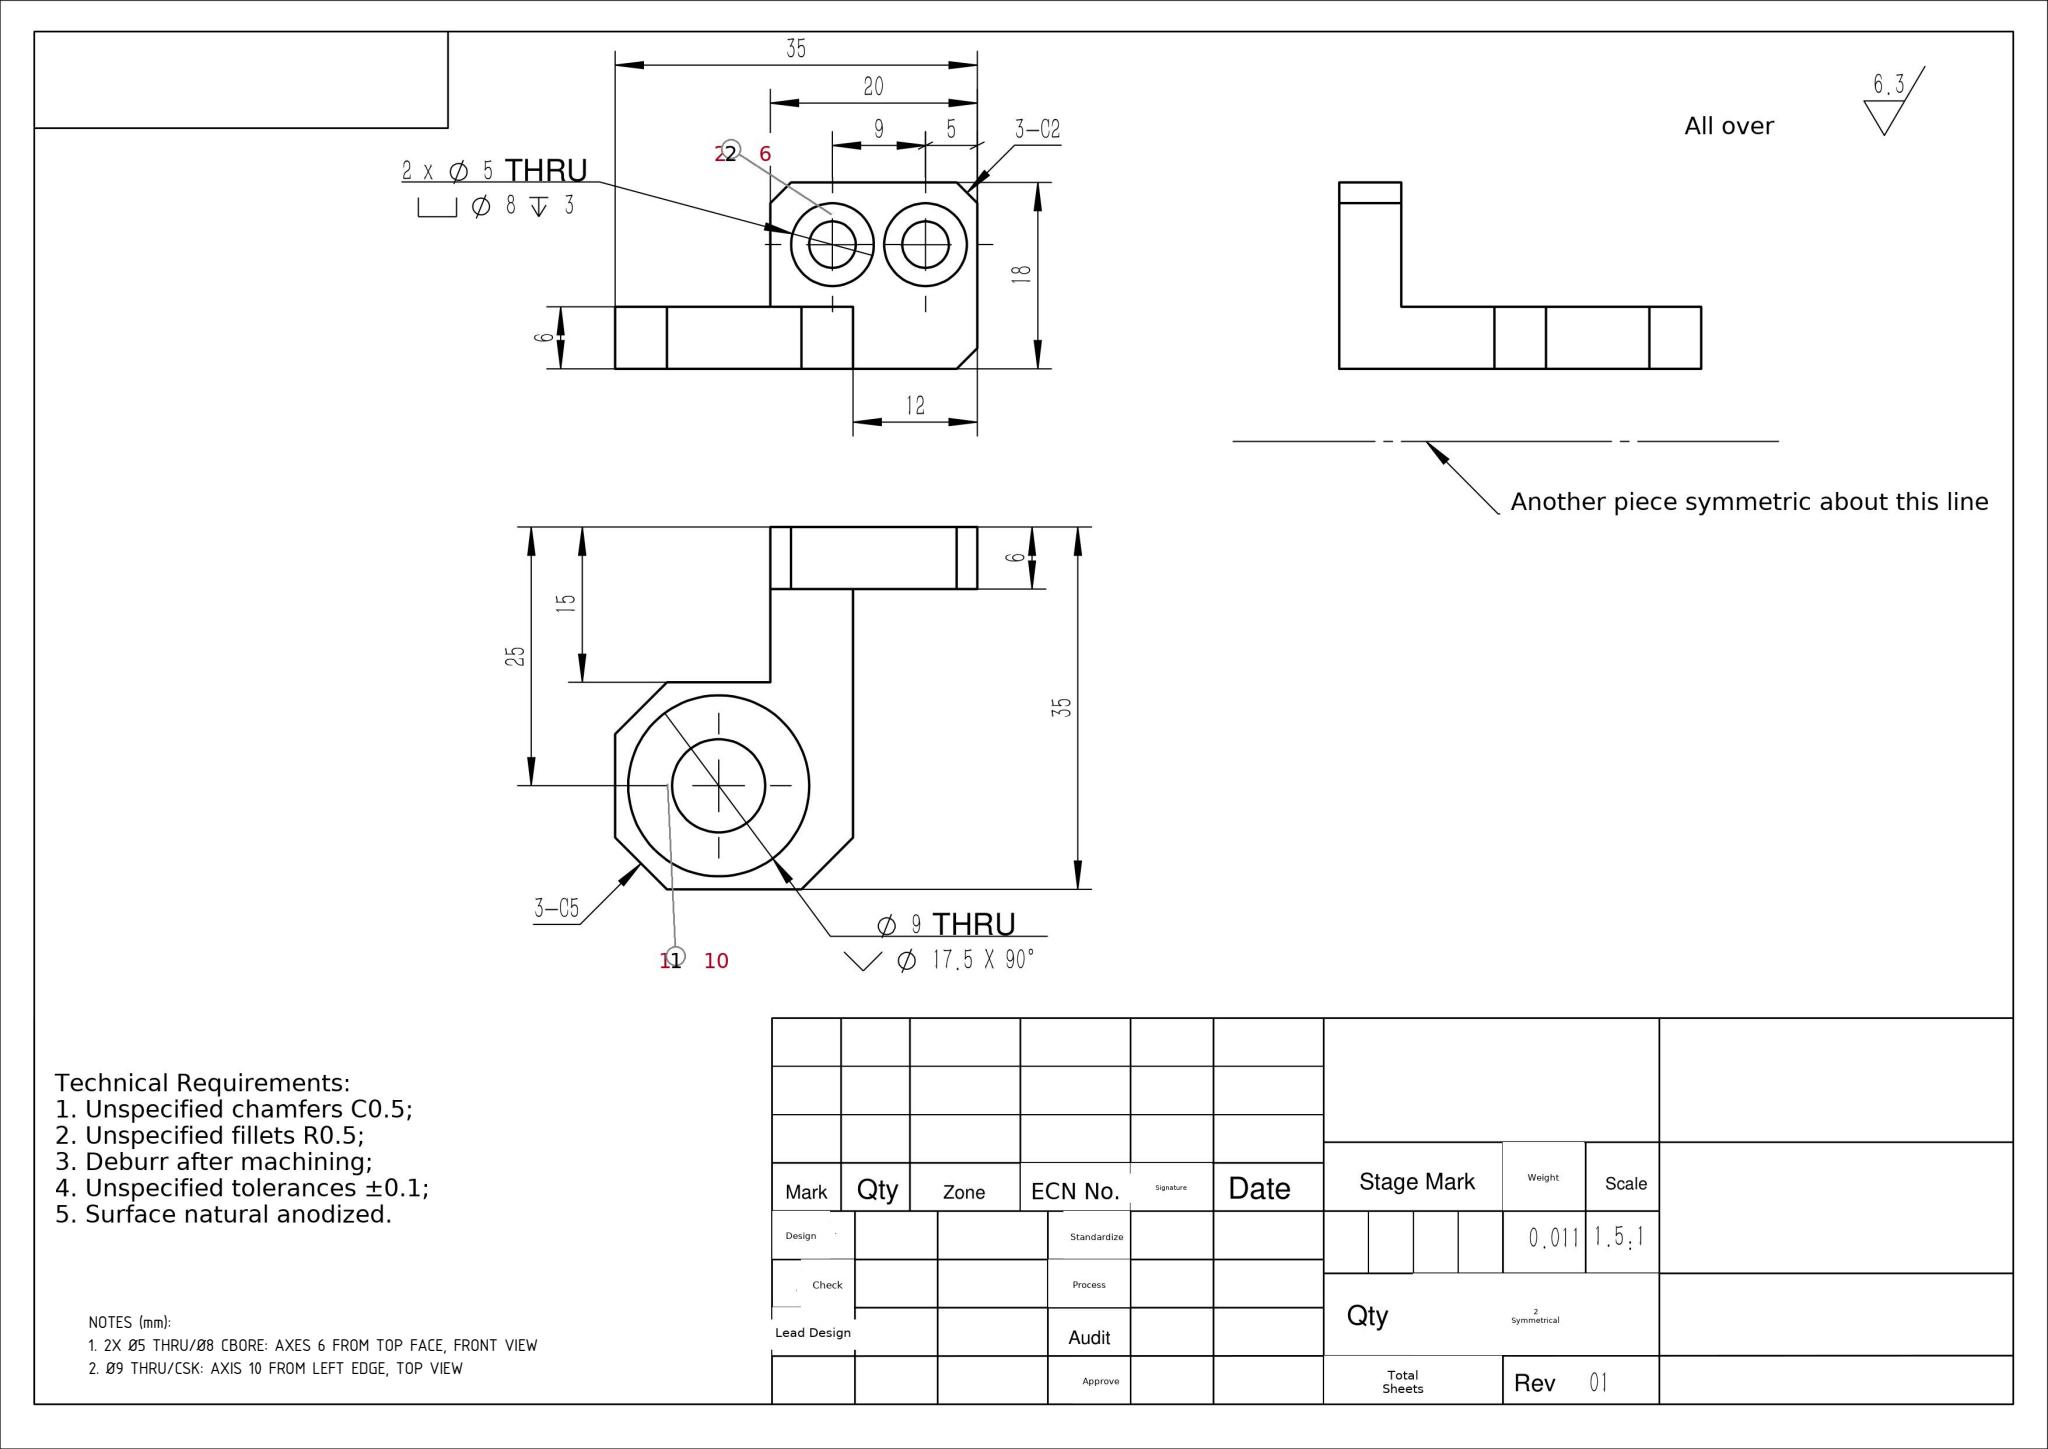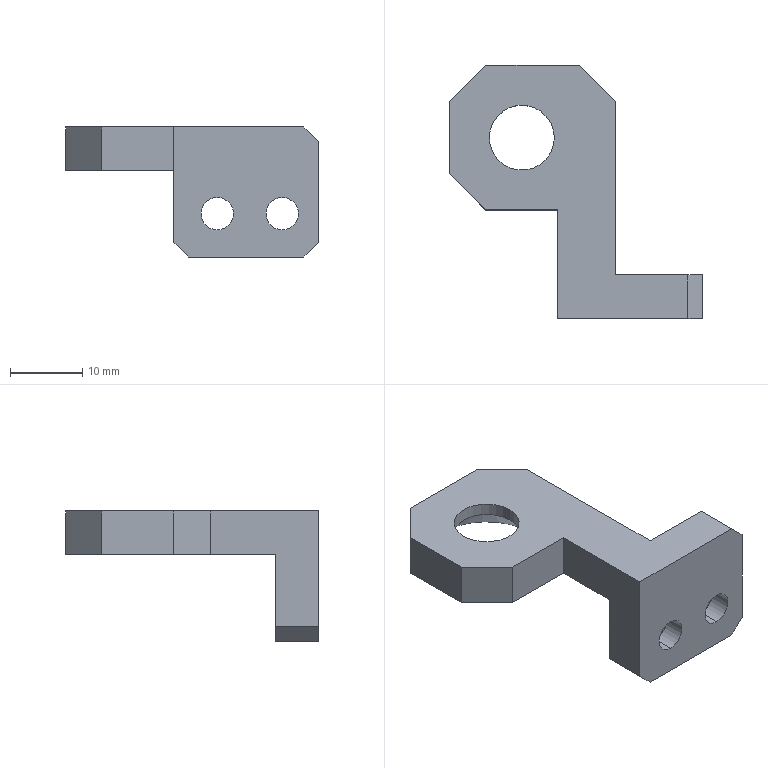Part | SolidWorks | mm | 1 solid | 31 faces | box 35 x 35 x 18 mm | volume 3977 mm3 | plane 19 | cylinder 10 | cone 2 | commonest cylinder face diameters 8 x4 4.5 x4 9 x2
Drawing notes:
2X Ø5 THRU/Ø8 CBORE: AXES 6 FROM TOP FACE, FRONT VIEW | from the solid: Y-axis cyls Ø5/Ø8 at z=6.0 of 18.0 bbox height; top face plane z=0
Ø9 THRU/CSK: AXIS 10 FROM LEFT EDGE, TOP VIEW | from the solid: Z-axis Ø9 cyl at x=10.0 (y=25.0) in 35.0 x 35.0 bbox; left edge plane x=0
build123d program:
from build123d import *

# Parameters (mm, degrees)
SKETCH1_W                                         = 35
SKETCH1_H                                         = 35
BOSS_EXTRUDE1_DEPTH                               = 6
SKETCH2_W                                         = 35
SKETCH2_H                                         = 12
BOSS_EXTRUDE2_DEPTH                               = 6
HOLE_SIZE_ACCORDING_TO_HEXAGON_SOCKET_D           = 4.5
HOLE_SIZE_ACCORDING_TO_HEXAGON_SOCKET_CBORE_D     = 8
HOLE_SIZE_ACCORDING_TO_HEXAGON_SOCKET_CBORE_DEPTH = 3
SKETCH7_W                                         = 15
SKETCH7_H                                         = 15
CUT_EXTRUDE1_DEPTH                                = 31.602
SKETCH8_W                                         = 12
SKETCH8_H                                         = 29
CUT_EXTRUDE2_DEPTH                                = 28.505
CHAMFER1_SIZE                                     = 5
CHAMFER2_SIZE                                     = 2


with BuildPart() as part:
    # Sketch1 → Boss-Extrude1 (new body)
    with BuildSketch(Plane.XY):
        Rectangle(SKETCH1_W, SKETCH1_H)
    extrude(amount=BOSS_EXTRUDE1_DEPTH)

    # Sketch2 → Boss-Extrude2 (add)
    with BuildSketch(Plane.XZ.offset(17.5)):
        with Locations((0, -6)):
            Rectangle(SKETCH2_W, SKETCH2_H)
    extrude(amount=-BOSS_EXTRUDE2_DEPTH)

    # Sketch3 → Hole Size _ according to Phillips_ Raise (revolve, cut)
    with BuildSketch(Plane(origin=(-7.5, 7.5, 0), x_dir=(0, 1, 0), z_dir=(1, 0, 0))):
        Polygon((0, 0), (0, 6), (4.5, 6), (4.5, 4.25), (8.75, 0), align=None)
    revolve(axis=Axis((-7.5, 7.5, -6.35), (0, 0, 1)), mode=Mode.SUBTRACT)

    # Hole Size _ according to_ Hexagon Socket (through all)
    with Locations(Plane(origin=(0, -11.5, 0), x_dir=(1, 0, 0), z_dir=(0, 1, 0))):
        with Locations((3.5, 6), (12.5, 6)):
            CounterBoreHole(HOLE_SIZE_ACCORDING_TO_HEXAGON_SOCKET_D / 2, HOLE_SIZE_ACCORDING_TO_HEXAGON_SOCKET_CBORE_D / 2, HOLE_SIZE_ACCORDING_TO_HEXAGON_SOCKET_CBORE_DEPTH)

    # Sketch7 → Cut-Extrude1 (cut, through all)
    with BuildSketch(Plane(origin=(0, 0, -12), x_dir=(-1, 0, 0), z_dir=(0, 0, -1))):
        with Locations((10, -10)):
            Rectangle(SKETCH7_W, SKETCH7_H)
    extrude(amount=-CUT_EXTRUDE1_DEPTH, mode=Mode.SUBTRACT)

    # Sketch8 → Cut-Extrude2 (cut, through all)
    with BuildSketch(Plane(origin=(0, 0, 0), x_dir=(-1, 0, 0), z_dir=(0, 0, -1))):
        with Locations((-11.5, 3)):
            Rectangle(SKETCH8_W, SKETCH8_H)
    extrude(amount=-CUT_EXTRUDE2_DEPTH, mode=Mode.SUBTRACT)

    # Chamfer1
    chamfer1_edges = [part.edges().sort_by_distance(p)[0] for p in [
        (-17.5, 17.5, 3),
        (-17.5, -2.5, 3),
        (5.5, 17.5, 3),
    ]]
    chamfer(chamfer1_edges, length=CHAMFER1_SIZE)

    # Chamfer2
    chamfer2_edges = [part.edges().sort_by_distance(p)[0] for p in [
        (17.5, -14.5, -12),
        (-2.5, -14.5, -12),
        (17.5, -14.5, 6),
    ]]
    chamfer(chamfer2_edges, length=CHAMFER2_SIZE)


solid = part.part
STEP:
#1=CARTESIAN_POINT('',(3.5,-14.5,-10.));
#2=VERTEX_POINT('',#1);
#3=CARTESIAN_POINT('',(3.5,-14.5,-2.));
#4=VERTEX_POINT('',#3);
#5=CARTESIAN_POINT('',(3.5,-14.5,-6.));
#6=DIRECTION('',(0.,1.,0.));
#7=DIRECTION('',(0.,0.,1.));
#8=AXIS2_PLACEMENT_3D('',#5,#6,#7);
#9=CIRCLE('',#8,4.);
#10=EDGE_CURVE('',#2,#4,#9,.T.);
#11=ORIENTED_EDGE('',*,*,#10,.F.);
#12=CARTESIAN_POINT('',(3.5,-11.5,-10.));
#13=VERTEX_POINT('',#12);
#14=CARTESIAN_POINT('',(3.5,-11.5,-10.));
#15=DIRECTION('',(0.,1.,0.));
#16=VECTOR('',#15,1000.);
#17=LINE('',#14,#16);
#18=EDGE_CURVE('',#2,#13,#17,.T.);
#19=ORIENTED_EDGE('',*,*,#18,.T.);
#20=CARTESIAN_POINT('',(3.5,-11.5,-2.));
#21=VERTEX_POINT('',#20);
#22=CARTESIAN_POINT('',(3.5,-11.5,-6.));
#23=DIRECTION('',(0.,1.,0.));
#24=DIRECTION('',(0.,0.,1.));
#25=AXIS2_PLACEMENT_3D('',#22,#23,#24);
#26=CIRCLE('',#25,4.);
#27=EDGE_CURVE('',#13,#21,#26,.T.);
#28=ORIENTED_EDGE('',*,*,#27,.T.);
#29=CARTESIAN_POINT('',(3.5,-11.5,-2.));
#30=DIRECTION('',(0.,1.,0.));
#31=VECTOR('',#30,1000.);
#32=LINE('',#29,#31);
#33=EDGE_CURVE('',#4,#21,#32,.T.);
#34=ORIENTED_EDGE('',*,*,#33,.F.);
#35=EDGE_LOOP('',(#11,#19,#28,#34));
#36=FACE_OUTER_BOUND('',#35,.T.);
#37=CARTESIAN_POINT('',(3.5,-11.5,-6.));
#38=DIRECTION('',(0.,1.,0.));
#39=DIRECTION('',(0.,0.,1.));
#40=AXIS2_PLACEMENT_3D('',#37,#38,#39);
#41=CYLINDRICAL_SURFACE('',#40,4.);
#42=ADVANCED_FACE('',(#36),#41,.F.);
#43=CARTESIAN_POINT('',(3.5,-17.5,-8.25));
#44=VERTEX_POINT('',#43);
#45=CARTESIAN_POINT('',(3.5,-17.5,-3.75));
#46=VERTEX_POINT('',#45);
#47=CARTESIAN_POINT('',(3.5,-17.5,-6.));
#48=DIRECTION('',(0.,1.,0.));
#49=DIRECTION('',(0.,0.,1.));
#50=AXIS2_PLACEMENT_3D('',#47,#48,#49);
#51=CIRCLE('',#50,2.25);
#52=EDGE_CURVE('',#44,#46,#51,.T.);
#53=ORIENTED_EDGE('',*,*,#52,.F.);
#54=CARTESIAN_POINT('',(3.5,-14.5,-8.25));
#55=VERTEX_POINT('',#54);
#56=CARTESIAN_POINT('',(3.5,-11.5,-8.25));
#57=DIRECTION('',(0.,1.,0.));
#58=VECTOR('',#57,1000.);
#59=LINE('',#56,#58);
#60=EDGE_CURVE('',#44,#55,#59,.T.);
#61=ORIENTED_EDGE('',*,*,#60,.T.);
#62=CARTESIAN_POINT('',(3.5,-14.5,-3.75));
#63=VERTEX_POINT('',#62);
#64=CARTESIAN_POINT('',(3.5,-14.5,-6.));
#65=DIRECTION('',(0.,1.,0.));
#66=DIRECTION('',(0.,0.,1.));
#67=AXIS2_PLACEMENT_3D('',#64,#65,#66);
#68=CIRCLE('',#67,2.25);
#69=EDGE_CURVE('',#55,#63,#68,.T.);
#70=ORIENTED_EDGE('',*,*,#69,.T.);
#71=CARTESIAN_POINT('',(3.5,-11.5,-3.75));
#72=DIRECTION('',(0.,1.,0.));
#73=VECTOR('',#72,1000.);
#74=LINE('',#71,#73);
#75=EDGE_CURVE('',#46,#63,#74,.T.);
#76=ORIENTED_EDGE('',*,*,#75,.F.);
#77=EDGE_LOOP('',(#53,#61,#70,#76));
#78=FACE_OUTER_BOUND('',#77,.T.);
#79=CARTESIAN_POINT('',(3.5,-11.5,-6.));
#80=DIRECTION('',(0.,1.,0.));
#81=DIRECTION('',(0.,0.,1.));
#82=AXIS2_PLACEMENT_3D('',#79,#80,#81);
#83=CYLINDRICAL_SURFACE('',#82,2.25);
#84=ADVANCED_FACE('',(#78),#83,.F.);
#85=CARTESIAN_POINT('',(12.5,-14.5,-10.));
#86=VERTEX_POINT('',#85);
#87=CARTESIAN_POINT('',(12.5,-14.5,-2.));
#88=VERTEX_POINT('',#87);
#89=CARTESIAN_POINT('',(12.5,-14.5,-6.));
#90=DIRECTION('',(0.,1.,0.));
#91=DIRECTION('',(0.,0.,1.));
#92=AXIS2_PLACEMENT_3D('',#89,#90,#91);
#93=CIRCLE('',#92,4.);
#94=EDGE_CURVE('',#86,#88,#93,.T.);
#95=ORIENTED_EDGE('',*,*,#94,.F.);
#96=CARTESIAN_POINT('',(12.5,-11.5,-10.));
#97=VERTEX_POINT('',#96);
#98=CARTESIAN_POINT('',(12.5,-11.5,-10.));
#99=DIRECTION('',(0.,1.,0.));
#100=VECTOR('',#99,1000.);
#101=LINE('',#98,#100);
#102=EDGE_CURVE('',#86,#97,#101,.T.);
#103=ORIENTED_EDGE('',*,*,#102,.T.);
#104=CARTESIAN_POINT('',(12.5,-11.5,-2.));
#105=VERTEX_POINT('',#104);
#106=CARTESIAN_POINT('',(12.5,-11.5,-6.));
#107=DIRECTION('',(0.,1.,0.));
#108=DIRECTION('',(0.,0.,1.));
#109=AXIS2_PLACEMENT_3D('',#106,#107,#108);
#110=CIRCLE('',#109,4.);
#111=EDGE_CURVE('',#97,#105,#110,.T.);
#112=ORIENTED_EDGE('',*,*,#111,.T.);
#113=CARTESIAN_POINT('',(12.5,-11.5,-2.));
#114=DIRECTION('',(0.,1.,0.));
#115=VECTOR('',#114,1000.);
#116=LINE('',#113,#115);
#117=EDGE_CURVE('',#88,#105,#116,.T.);
#118=ORIENTED_EDGE('',*,*,#117,.F.);
#119=EDGE_LOOP('',(#95,#103,#112,#118));
#120=FACE_OUTER_BOUND('',#119,.T.);
#121=CARTESIAN_POINT('',(12.5,-11.5,-6.));
#122=DIRECTION('',(0.,1.,0.));
#123=DIRECTION('',(0.,0.,1.));
#124=AXIS2_PLACEMENT_3D('',#121,#122,#123);
#125=CYLINDRICAL_SURFACE('',#124,4.);
#126=ADVANCED_FACE('',(#120),#125,.F.);
#127=CARTESIAN_POINT('',(12.5,-17.5,-8.25));
#128=VERTEX_POINT('',#127);
#129=CARTESIAN_POINT('',(12.5,-17.5,-3.75));
#130=VERTEX_POINT('',#129);
#131=CARTESIAN_POINT('',(12.5,-17.5,-6.));
#132=DIRECTION('',(0.,1.,0.));
#133=DIRECTION('',(0.,0.,1.));
#134=AXIS2_PLACEMENT_3D('',#131,#132,#133);
#135=CIRCLE('',#134,2.25);
#136=EDGE_CURVE('',#128,#130,#135,.T.);
#137=ORIENTED_EDGE('',*,*,#136,.F.);
#138=CARTESIAN_POINT('',(12.5,-14.5,-8.25));
#139=VERTEX_POINT('',#138);
#140=CARTESIAN_POINT('',(12.5,-11.5,-8.25));
#141=DIRECTION('',(0.,1.,0.));
#142=VECTOR('',#141,1000.);
#143=LINE('',#140,#142);
#144=EDGE_CURVE('',#128,#139,#143,.T.);
#145=ORIENTED_EDGE('',*,*,#144,.T.);
#146=CARTESIAN_POINT('',(12.5,-14.5,-3.75));
#147=VERTEX_POINT('',#146);
#148=CARTESIAN_POINT('',(12.5,-14.5,-6.));
#149=DIRECTION('',(0.,1.,0.));
#150=DIRECTION('',(0.,0.,1.));
#151=AXIS2_PLACEMENT_3D('',#148,#149,#150);
#152=CIRCLE('',#151,2.25);
#153=EDGE_CURVE('',#139,#147,#152,.T.);
#154=ORIENTED_EDGE('',*,*,#153,.T.);
#155=CARTESIAN_POINT('',(12.5,-11.5,-3.75));
#156=DIRECTION('',(0.,1.,0.));
#157=VECTOR('',#156,1000.);
#158=LINE('',#155,#157);
#159=EDGE_CURVE('',#130,#147,#158,.T.);
#160=ORIENTED_EDGE('',*,*,#159,.F.);
#161=EDGE_LOOP('',(#137,#145,#154,#160));
#162=FACE_OUTER_BOUND('',#161,.T.);
#163=CARTESIAN_POINT('',(12.5,-11.5,-6.));
#164=DIRECTION('',(0.,1.,0.));
#165=DIRECTION('',(0.,0.,1.));
#166=AXIS2_PLACEMENT_3D('',#163,#164,#165);
#167=CYLINDRICAL_SURFACE('',#166,2.25);
#168=ADVANCED_FACE('',(#162),#167,.F.);
#169=CARTESIAN_POINT('',(-3.,7.5,4.25));
#170=VERTEX_POINT('',#169);
#171=CARTESIAN_POINT('',(-12.,7.5,4.25));
#172=VERTEX_POINT('',#171);
#173=CARTESIAN_POINT('',(-7.5,7.5,4.25));
#174=DIRECTION('',(0.,0.,-1.));
#175=DIRECTION('',(-1.,0.,0.));
#176=AXIS2_PLACEMENT_3D('',#173,#174,#175);
#177=CIRCLE('',#176,4.5);
#178=EDGE_CURVE('',#170,#172,#177,.T.);
#179=ORIENTED_EDGE('',*,*,#178,.F.);
#180=CARTESIAN_POINT('',(1.25,7.5,-0.));
#181=VERTEX_POINT('',#180);
#182=CARTESIAN_POINT('',(1.25,7.5,-0.));
#183=DIRECTION('',(0.7071,0.,-0.7071));
#184=VECTOR('',#183,1000.);
#185=LINE('',#182,#184);
#186=EDGE_CURVE('',#170,#181,#185,.T.);
#187=ORIENTED_EDGE('',*,*,#186,.T.);
#188=CARTESIAN_POINT('',(-16.25,7.5,-0.));
#189=VERTEX_POINT('',#188);
#190=CARTESIAN_POINT('',(-7.5,7.5,-0.));
#191=DIRECTION('',(0.,0.,-1.));
#192=DIRECTION('',(-1.,0.,0.));
#193=AXIS2_PLACEMENT_3D('',#190,#191,#192);
#194=CIRCLE('',#193,8.75);
#195=EDGE_CURVE('',#181,#189,#194,.T.);
#196=ORIENTED_EDGE('',*,*,#195,.T.);
#197=CARTESIAN_POINT('',(-16.25,7.5,-0.));
#198=DIRECTION('',(-0.7071,0.,-0.7071));
#199=VECTOR('',#198,1000.);
#200=LINE('',#197,#199);
#201=EDGE_CURVE('',#172,#189,#200,.T.);
#202=ORIENTED_EDGE('',*,*,#201,.F.);
#203=EDGE_LOOP('',(#179,#187,#196,#202));
#204=FACE_OUTER_BOUND('',#203,.T.);
#205=CARTESIAN_POINT('',(-7.5,7.5,-0.));
#206=DIRECTION('',(0.,0.,-1.));
#207=DIRECTION('',(-1.,0.,0.));
#208=AXIS2_PLACEMENT_3D('',#205,#206,#207);
#209=CONICAL_SURFACE('',#208,8.75,0.7854);
#210=ADVANCED_FACE('',(#204),#209,.F.);
#211=CARTESIAN_POINT('',(-3.,7.5,6.));
#212=VERTEX_POINT('',#211);
#213=CARTESIAN_POINT('',(-12.,7.5,6.));
#214=VERTEX_POINT('',#213);
#215=CARTESIAN_POINT('',(-7.5,7.5,6.));
#216=DIRECTION('',(0.,0.,-1.));
#217=DIRECTION('',(-1.,0.,0.));
#218=AXIS2_PLACEMENT_3D('',#215,#216,#217);
#219=CIRCLE('',#218,4.5);
#220=EDGE_CURVE('',#212,#214,#219,.T.);
#221=ORIENTED_EDGE('',*,*,#220,.F.);
#222=CARTESIAN_POINT('',(-3.,7.5,0.));
#223=DIRECTION('',(0.,0.,-1.));
#224=VECTOR('',#223,1000.);
#225=LINE('',#222,#224);
#226=EDGE_CURVE('',#212,#170,#225,.T.);
#227=ORIENTED_EDGE('',*,*,#226,.T.);
#228=ORIENTED_EDGE('',*,*,#178,.T.);
#229=CARTESIAN_POINT('',(-12.,7.5,0.));
#230=DIRECTION('',(0.,0.,-1.));
#231=VECTOR('',#230,1000.);
#232=LINE('',#229,#231);
#233=EDGE_CURVE('',#214,#172,#232,.T.);
#234=ORIENTED_EDGE('',*,*,#233,.F.);
#235=EDGE_LOOP('',(#221,#227,#228,#234));
#236=FACE_OUTER_BOUND('',#235,.T.);
#237=CARTESIAN_POINT('',(-7.5,7.5,0.));
#238=DIRECTION('',(0.,0.,-1.));
#239=DIRECTION('',(-1.,0.,0.));
#240=AXIS2_PLACEMENT_3D('',#237,#238,#239);
#241=CYLINDRICAL_SURFACE('',#240,4.5);
#242=ADVANCED_FACE('',(#236),#241,.F.);
#243=CARTESIAN_POINT('',(-17.5,12.5,0.));
#244=VERTEX_POINT('',#243);
#245=CARTESIAN_POINT('',(-17.5,2.5,0.));
#246=VERTEX_POINT('',#245);
#247=CARTESIAN_POINT('',(-17.5,-17.5,0.));
#248=DIRECTION('',(0.,-1.,0.));
#249=VECTOR('',#248,1000.);
#250=LINE('',#247,#249);
#251=EDGE_CURVE('',#244,#246,#250,.T.);
#252=ORIENTED_EDGE('',*,*,#251,.T.);
#253=CARTESIAN_POINT('',(-17.5,2.5,6.));
#254=VERTEX_POINT('',#253);
#255=CARTESIAN_POINT('',(-17.5,2.5,6.));
#256=DIRECTION('',(0.,0.,1.));
#257=VECTOR('',#256,1000.);
#258=LINE('',#255,#257);
#259=EDGE_CURVE('',#246,#254,#258,.T.);
#260=ORIENTED_EDGE('',*,*,#259,.T.);
#261=CARTESIAN_POINT('',(-17.5,12.5,6.));
#262=VERTEX_POINT('',#261);
#263=CARTESIAN_POINT('',(-17.5,-17.5,6.));
#264=DIRECTION('',(0.,-1.,0.));
#265=VECTOR('',#264,1000.);
#266=LINE('',#263,#265);
#267=EDGE_CURVE('',#262,#254,#266,.T.);
#268=ORIENTED_EDGE('',*,*,#267,.F.);
#269=CARTESIAN_POINT('',(-17.5,12.5,6.));
#270=DIRECTION('',(0.,0.,-1.));
#271=VECTOR('',#270,1000.);
#272=LINE('',#269,#271);
#273=EDGE_CURVE('',#262,#244,#272,.T.);
#274=ORIENTED_EDGE('',*,*,#273,.T.);
#275=EDGE_LOOP('',(#252,#260,#268,#274));
#276=FACE_OUTER_BOUND('',#275,.T.);
#277=CARTESIAN_POINT('',(-17.5,-17.5,6.));
#278=DIRECTION('',(1.,0.,0.));
#279=DIRECTION('',(0.,0.,-1.));
#280=AXIS2_PLACEMENT_3D('',#277,#278,#279);
#281=PLANE('',#280);
#282=ADVANCED_FACE('',(#276),#281,.F.);
#283=CARTESIAN_POINT('',(3.5,-17.5,-6.));
#284=DIRECTION('',(0.,1.,0.));
#285=DIRECTION('',(0.,0.,1.));
#286=AXIS2_PLACEMENT_3D('',#283,#284,#285);
#287=CIRCLE('',#286,2.25);
#288=EDGE_CURVE('',#46,#44,#287,.T.);
#289=ORIENTED_EDGE('',*,*,#288,.T.);
#290=ORIENTED_EDGE('',*,*,#52,.T.);
#291=EDGE_LOOP('',(#289,#290));
#292=FACE_BOUND('',#291,.T.);
#293=CARTESIAN_POINT('',(12.5,-17.5,-6.));
#294=DIRECTION('',(0.,1.,0.));
#295=DIRECTION('',(0.,0.,1.));
#296=AXIS2_PLACEMENT_3D('',#293,#294,#295);
#297=CIRCLE('',#296,2.25);
#298=EDGE_CURVE('',#130,#128,#297,.T.);
#299=ORIENTED_EDGE('',*,*,#298,.T.);
#300=ORIENTED_EDGE('',*,*,#136,.T.);
#301=EDGE_LOOP('',(#299,#300));
#302=FACE_BOUND('',#301,.T.);
#303=CARTESIAN_POINT('',(17.5,-17.5,4.));
#304=VERTEX_POINT('',#303);
#305=CARTESIAN_POINT('',(17.5,-17.5,-10.));
#306=VERTEX_POINT('',#305);
#307=CARTESIAN_POINT('',(17.5,-17.5,6.));
#308=DIRECTION('',(0.,0.,-1.));
#309=VECTOR('',#308,1000.);
#310=LINE('',#307,#309);
#311=EDGE_CURVE('',#304,#306,#310,.T.);
#312=ORIENTED_EDGE('',*,*,#311,.F.);
#313=CARTESIAN_POINT('',(15.5,-17.5,6.));
#314=VERTEX_POINT('',#313);
#315=CARTESIAN_POINT('',(15.5,-17.5,6.));
#316=DIRECTION('',(-0.7071,0.,0.7071));
#317=VECTOR('',#316,1000.);
#318=LINE('',#315,#317);
#319=EDGE_CURVE('',#304,#314,#318,.T.);
#320=ORIENTED_EDGE('',*,*,#319,.T.);
#321=CARTESIAN_POINT('',(-2.5,-17.5,6.));
#322=VERTEX_POINT('',#321);
#323=CARTESIAN_POINT('',(17.5,-17.5,6.));
#324=DIRECTION('',(1.,0.,0.));
#325=VECTOR('',#324,1000.);
#326=LINE('',#323,#325);
#327=EDGE_CURVE('',#322,#314,#326,.T.);
#328=ORIENTED_EDGE('',*,*,#327,.F.);
#329=CARTESIAN_POINT('',(-2.5,-17.5,-10.));
#330=VERTEX_POINT('',#329);
#331=CARTESIAN_POINT('',(-2.5,-17.5,6.));
#332=DIRECTION('',(0.,0.,-1.));
#333=VECTOR('',#332,1000.);
#334=LINE('',#331,#333);
#335=EDGE_CURVE('',#322,#330,#334,.T.);
#336=ORIENTED_EDGE('',*,*,#335,.T.);
#337=CARTESIAN_POINT('',(-0.5,-17.5,-12.));
#338=VERTEX_POINT('',#337);
#339=CARTESIAN_POINT('',(-2.5,-17.5,-10.));
#340=DIRECTION('',(0.7071,0.,-0.7071));
#341=VECTOR('',#340,1000.);
#342=LINE('',#339,#341);
#343=EDGE_CURVE('',#330,#338,#342,.T.);
#344=ORIENTED_EDGE('',*,*,#343,.T.);
#345=CARTESIAN_POINT('',(15.5,-17.5,-12.));
#346=VERTEX_POINT('',#345);
#347=CARTESIAN_POINT('',(-17.5,-17.5,-12.));
#348=DIRECTION('',(1.,0.,0.));
#349=VECTOR('',#348,1000.);
#350=LINE('',#347,#349);
#351=EDGE_CURVE('',#338,#346,#350,.T.);
#352=ORIENTED_EDGE('',*,*,#351,.T.);
#353=CARTESIAN_POINT('',(15.5,-17.5,-12.));
#354=DIRECTION('',(0.7071,0.,0.7071));
#355=VECTOR('',#354,1000.);
#356=LINE('',#353,#355);
#357=EDGE_CURVE('',#346,#306,#356,.T.);
#358=ORIENTED_EDGE('',*,*,#357,.T.);
#359=EDGE_LOOP('',(#312,#320,#328,#336,#344,#352,#358));
#360=FACE_OUTER_BOUND('',#359,.T.);
#361=CARTESIAN_POINT('',(17.5,-17.5,6.));
#362=DIRECTION('',(0.,1.,0.));
#363=DIRECTION('',(0.,0.,1.));
#364=AXIS2_PLACEMENT_3D('',#361,#362,#363);
#365=PLANE('',#364);
#366=ADVANCED_FACE('',(#292,#302,#360),#365,.F.);
#367=CARTESIAN_POINT('',(17.5,-11.5,-10.));
#368=VERTEX_POINT('',#367);
#369=CARTESIAN_POINT('',(17.5,-11.5,4.));
#370=VERTEX_POINT('',#369);
#371=CARTESIAN_POINT('',(17.5,-11.5,0.));
#372=DIRECTION('',(0.,0.,1.));
#373=VECTOR('',#372,1000.);
#374=LINE('',#371,#373);
#375=EDGE_CURVE('',#368,#370,#374,.T.);
#376=ORIENTED_EDGE('',*,*,#375,.T.);
#377=CARTESIAN_POINT('',(17.5,-17.5,4.));
#378=DIRECTION('',(0.,-1.,0.));
#379=VECTOR('',#378,1000.);
#380=LINE('',#377,#379);
#381=EDGE_CURVE('',#370,#304,#380,.T.);
#382=ORIENTED_EDGE('',*,*,#381,.T.);
#383=ORIENTED_EDGE('',*,*,#311,.T.);
#384=CARTESIAN_POINT('',(17.5,-11.5,-10.));
#385=DIRECTION('',(0.,1.,0.));
#386=VECTOR('',#385,1000.);
#387=LINE('',#384,#386);
#388=EDGE_CURVE('',#306,#368,#387,.T.);
#389=ORIENTED_EDGE('',*,*,#388,.T.);
#390=EDGE_LOOP('',(#376,#382,#383,#389));
#391=FACE_OUTER_BOUND('',#390,.T.);
#392=CARTESIAN_POINT('',(17.5,-17.5,6.));
#393=DIRECTION('',(-1.,0.,0.));
#394=DIRECTION('',(0.,0.,1.));
#395=AXIS2_PLACEMENT_3D('',#392,#393,#394);
#396=PLANE('',#395);
#397=ADVANCED_FACE('',(#391),#396,.F.);
#398=CARTESIAN_POINT('',(0.5,17.5,6.));
#399=VERTEX_POINT('',#398);
#400=CARTESIAN_POINT('',(-12.5,17.5,6.));
#401=VERTEX_POINT('',#400);
#402=CARTESIAN_POINT('',(17.5,17.5,6.));
#403=DIRECTION('',(-1.,-0.,0.));
#404=VECTOR('',#403,1000.);
#405=LINE('',#402,#404);
#406=EDGE_CURVE('',#399,#401,#405,.T.);
#407=ORIENTED_EDGE('',*,*,#406,.F.);
#408=CARTESIAN_POINT('',(0.5,17.5,0.));
#409=VERTEX_POINT('',#408);
#410=CARTESIAN_POINT('',(0.5,17.5,6.));
#411=DIRECTION('',(0.,0.,-1.));
#412=VECTOR('',#411,1000.);
#413=LINE('',#410,#412);
#414=EDGE_CURVE('',#399,#409,#413,.T.);
#415=ORIENTED_EDGE('',*,*,#414,.T.);
#416=CARTESIAN_POINT('',(-12.5,17.5,0.));
#417=VERTEX_POINT('',#416);
#418=CARTESIAN_POINT('',(17.5,17.5,0.));
#419=DIRECTION('',(-1.,-0.,0.));
#420=VECTOR('',#419,1000.);
#421=LINE('',#418,#420);
#422=EDGE_CURVE('',#409,#417,#421,.T.);
#423=ORIENTED_EDGE('',*,*,#422,.T.);
#424=CARTESIAN_POINT('',(-12.5,17.5,6.));
#425=DIRECTION('',(0.,0.,1.));
#426=VECTOR('',#425,1000.);
#427=LINE('',#424,#426);
#428=EDGE_CURVE('',#417,#401,#427,.T.);
#429=ORIENTED_EDGE('',*,*,#428,.T.);
#430=EDGE_LOOP('',(#407,#415,#423,#429));
#431=FACE_OUTER_BOUND('',#430,.T.);
#432=CARTESIAN_POINT('',(17.5,17.5,6.));
#433=DIRECTION('',(0.,-1.,0.));
#434=DIRECTION('',(1.,0.,0.));
#435=AXIS2_PLACEMENT_3D('',#432,#433,#434);
#436=PLANE('',#435);
#437=ADVANCED_FACE('',(#431),#436,.F.);
#438=ORIENTED_EDGE('',*,*,#327,.T.);
#439=CARTESIAN_POINT('',(15.5,-11.5,6.));
#440=VERTEX_POINT('',#439);
#441=CARTESIAN_POINT('',(15.5,-11.5,6.));
#442=DIRECTION('',(0.,1.,0.));
#443=VECTOR('',#442,1000.);
#444=LINE('',#441,#443);
#445=EDGE_CURVE('',#314,#440,#444,.T.);
#446=ORIENTED_EDGE('',*,*,#445,.T.);
#447=CARTESIAN_POINT('',(5.5,-11.5,6.));
#448=VERTEX_POINT('',#447);
#449=CARTESIAN_POINT('',(17.5,-11.5,6.));
#450=DIRECTION('',(-1.,0.,0.));
#451=VECTOR('',#450,1000.);
#452=LINE('',#449,#451);
#453=EDGE_CURVE('',#440,#448,#452,.T.);
#454=ORIENTED_EDGE('',*,*,#453,.T.);
#455=CARTESIAN_POINT('',(5.5,12.5,6.));
#456=VERTEX_POINT('',#455);
#457=CARTESIAN_POINT('',(5.5,17.5,6.));
#458=DIRECTION('',(0.,1.,0.));
#459=VECTOR('',#458,1000.);
#460=LINE('',#457,#459);
#461=EDGE_CURVE('',#448,#456,#460,.T.);
#462=ORIENTED_EDGE('',*,*,#461,.T.);
#463=CARTESIAN_POINT('',(9.,9.,6.));
#464=DIRECTION('',(-0.7071,0.7071,0.));
#465=VECTOR('',#464,1000.);
#466=LINE('',#463,#465);
#467=EDGE_CURVE('',#456,#399,#466,.T.);
#468=ORIENTED_EDGE('',*,*,#467,.T.);
#469=ORIENTED_EDGE('',*,*,#406,.T.);
#470=CARTESIAN_POINT('',(-15.,15.,6.));
#471=DIRECTION('',(-0.7071,-0.7071,0.));
#472=VECTOR('',#471,1000.);
#473=LINE('',#470,#472);
#474=EDGE_CURVE('',#401,#262,#473,.T.);
#475=ORIENTED_EDGE('',*,*,#474,.T.);
#476=ORIENTED_EDGE('',*,*,#267,.T.);
#477=CARTESIAN_POINT('',(-12.5,-2.5,6.));
#478=VERTEX_POINT('',#477);
#479=CARTESIAN_POINT('',(-7.5,-7.5,6.));
#480=DIRECTION('',(0.7071,-0.7071,0.));
#481=VECTOR('',#480,1000.);
#482=LINE('',#479,#481);
#483=EDGE_CURVE('',#254,#478,#482,.T.);
#484=ORIENTED_EDGE('',*,*,#483,.T.);
#485=CARTESIAN_POINT('',(-2.5,-2.5,6.));
#486=VERTEX_POINT('',#485);
#487=CARTESIAN_POINT('',(-17.5,-2.5,6.));
#488=DIRECTION('',(1.,-0.,0.));
#489=VECTOR('',#488,1000.);
#490=LINE('',#487,#489);
#491=EDGE_CURVE('',#478,#486,#490,.T.);
#492=ORIENTED_EDGE('',*,*,#491,.T.);
#493=CARTESIAN_POINT('',(-2.5,-17.5,6.));
#494=DIRECTION('',(0.,-1.,0.));
#495=VECTOR('',#494,1000.);
#496=LINE('',#493,#495);
#497=EDGE_CURVE('',#486,#322,#496,.T.);
#498=ORIENTED_EDGE('',*,*,#497,.T.);
#499=EDGE_LOOP('',(#438,#446,#454,#462,#468,#469,#475,#476,#484,#492,#498));
#500=FACE_OUTER_BOUND('',#499,.T.);
#501=CARTESIAN_POINT('',(-7.5,7.5,6.));
#502=DIRECTION('',(0.,0.,-1.));
#503=DIRECTION('',(-1.,0.,0.));
#504=AXIS2_PLACEMENT_3D('',#501,#502,#503);
#505=CIRCLE('',#504,4.5);
#506=EDGE_CURVE('',#214,#212,#505,.T.);
#507=ORIENTED_EDGE('',*,*,#506,.T.);
#508=ORIENTED_EDGE('',*,*,#220,.T.);
#509=EDGE_LOOP('',(#507,#508));
#510=FACE_BOUND('',#509,.T.);
#511=CARTESIAN_POINT('',(0.,0.,6.));
#512=DIRECTION('',(0.,0.,1.));
#513=DIRECTION('',(1.,0.,0.));
#514=AXIS2_PLACEMENT_3D('',#511,#512,#513);
#515=PLANE('',#514);
#516=ADVANCED_FACE('',(#500,#510),#515,.T.);
#517=CARTESIAN_POINT('',(-7.5,7.5,-0.));
#518=DIRECTION('',(0.,0.,-1.));
#519=DIRECTION('',(-1.,0.,0.));
#520=AXIS2_PLACEMENT_3D('',#517,#518,#519);
#521=CIRCLE('',#520,8.75);
#522=EDGE_CURVE('',#189,#181,#521,.T.);
#523=ORIENTED_EDGE('',*,*,#522,.F.);
#524=ORIENTED_EDGE('',*,*,#195,.F.);
#525=EDGE_LOOP('',(#523,#524));
#526=FACE_BOUND('',#525,.T.);
#527=ORIENTED_EDGE('',*,*,#422,.F.);
#528=CARTESIAN_POINT('',(5.5,12.5,0.));
#529=VERTEX_POINT('',#528);
#530=CARTESIAN_POINT('',(0.5,17.5,0.));
#531=DIRECTION('',(0.7071,-0.7071,0.));
#532=VECTOR('',#531,1000.);
#533=LINE('',#530,#532);
#534=EDGE_CURVE('',#409,#529,#533,.T.);
#535=ORIENTED_EDGE('',*,*,#534,.T.);
#536=CARTESIAN_POINT('',(5.5,-11.5,0.));
#537=VERTEX_POINT('',#536);
#538=CARTESIAN_POINT('',(5.5,17.5,0.));
#539=DIRECTION('',(0.,1.,0.));
#540=VECTOR('',#539,1000.);
#541=LINE('',#538,#540);
#542=EDGE_CURVE('',#537,#529,#541,.T.);
#543=ORIENTED_EDGE('',*,*,#542,.F.);
#544=CARTESIAN_POINT('',(-2.5,-11.5,0.));
#545=VERTEX_POINT('',#544);
#546=CARTESIAN_POINT('',(-17.5,-11.5,0.));
#547=DIRECTION('',(-1.,-0.,0.));
#548=VECTOR('',#547,1000.);
#549=LINE('',#546,#548);
#550=EDGE_CURVE('',#537,#545,#549,.T.);
#551=ORIENTED_EDGE('',*,*,#550,.T.);
#552=CARTESIAN_POINT('',(-2.5,-2.5,0.));
#553=VERTEX_POINT('',#552);
#554=CARTESIAN_POINT('',(-2.5,0.,0.));
#555=DIRECTION('',(0.,1.,0.));
#556=VECTOR('',#555,1000.);
#557=LINE('',#554,#556);
#558=EDGE_CURVE('',#545,#553,#557,.T.);
#559=ORIENTED_EDGE('',*,*,#558,.T.);
#560=CARTESIAN_POINT('',(-12.5,-2.5,0.));
#561=VERTEX_POINT('',#560);
#562=CARTESIAN_POINT('',(-0.,-2.5,0.));
#563=DIRECTION('',(-1.,0.,0.));
#564=VECTOR('',#563,1000.);
#565=LINE('',#562,#564);
#566=EDGE_CURVE('',#553,#561,#565,.T.);
#567=ORIENTED_EDGE('',*,*,#566,.T.);
#568=CARTESIAN_POINT('',(-12.5,-2.5,0.));
#569=DIRECTION('',(-0.7071,0.7071,0.));
#570=VECTOR('',#569,1000.);
#571=LINE('',#568,#570);
#572=EDGE_CURVE('',#561,#246,#571,.T.);
#573=ORIENTED_EDGE('',*,*,#572,.T.);
#574=ORIENTED_EDGE('',*,*,#251,.F.);
#575=CARTESIAN_POINT('',(-17.5,12.5,0.));
#576=DIRECTION('',(0.7071,0.7071,0.));
#577=VECTOR('',#576,1000.);
#578=LINE('',#575,#577);
#579=EDGE_CURVE('',#244,#417,#578,.T.);
#580=ORIENTED_EDGE('',*,*,#579,.T.);
#581=EDGE_LOOP('',(#527,#535,#543,#551,#559,#567,#573,#574,#580));
#582=FACE_OUTER_BOUND('',#581,.T.);
#583=CARTESIAN_POINT('',(0.,0.,0.));
#584=DIRECTION('',(0.,0.,1.));
#585=DIRECTION('',(1.,0.,0.));
#586=AXIS2_PLACEMENT_3D('',#583,#584,#585);
#587=PLANE('',#586);
#588=ADVANCED_FACE('',(#526,#582),#587,.F.);
#589=ORIENTED_EDGE('',*,*,#351,.F.);
#590=CARTESIAN_POINT('',(-0.5,-11.5,-12.));
#591=VERTEX_POINT('',#590);
#592=CARTESIAN_POINT('',(-0.5,-11.5,-12.));
#593=DIRECTION('',(0.,1.,0.));
#594=VECTOR('',#593,1000.);
#595=LINE('',#592,#594);
#596=EDGE_CURVE('',#338,#591,#595,.T.);
#597=ORIENTED_EDGE('',*,*,#596,.T.);
#598=CARTESIAN_POINT('',(15.5,-11.5,-12.));
#599=VERTEX_POINT('',#598);
#600=CARTESIAN_POINT('',(-17.5,-11.5,-12.));
#601=DIRECTION('',(1.,0.,0.));
#602=VECTOR('',#601,1000.);
#603=LINE('',#600,#602);
#604=EDGE_CURVE('',#591,#599,#603,.T.);
#605=ORIENTED_EDGE('',*,*,#604,.T.);
#606=CARTESIAN_POINT('',(15.5,-17.5,-12.));
#607=DIRECTION('',(0.,-1.,0.));
#608=VECTOR('',#607,1000.);
#609=LINE('',#606,#608);
#610=EDGE_CURVE('',#599,#346,#609,.T.);
#611=ORIENTED_EDGE('',*,*,#610,.T.);
#612=EDGE_LOOP('',(#589,#597,#605,#611));
#613=FACE_OUTER_BOUND('',#612,.T.);
#614=CARTESIAN_POINT('',(-17.5,-11.5,-12.));
#615=DIRECTION('',(0.,0.,-1.));
#616=DIRECTION('',(-1.,0.,0.));
#617=AXIS2_PLACEMENT_3D('',#614,#615,#616);
#618=PLANE('',#617);
#619=ADVANCED_FACE('',(#613),#618,.T.);
#620=CARTESIAN_POINT('',(3.5,-11.5,-6.));
#621=DIRECTION('',(0.,1.,0.));
#622=DIRECTION('',(0.,0.,1.));
#623=AXIS2_PLACEMENT_3D('',#620,#621,#622);
#624=CIRCLE('',#623,4.);
#625=EDGE_CURVE('',#21,#13,#624,.T.);
#626=ORIENTED_EDGE('',*,*,#625,.F.);
#627=ORIENTED_EDGE('',*,*,#27,.F.);
#628=EDGE_LOOP('',(#626,#627));
#629=FACE_BOUND('',#628,.T.);
#630=CARTESIAN_POINT('',(12.5,-11.5,-6.));
#631=DIRECTION('',(0.,1.,0.));
#632=DIRECTION('',(0.,0.,1.));
#633=AXIS2_PLACEMENT_3D('',#630,#631,#632);
#634=CIRCLE('',#633,4.);
#635=EDGE_CURVE('',#105,#97,#634,.T.);
#636=ORIENTED_EDGE('',*,*,#635,.F.);
#637=ORIENTED_EDGE('',*,*,#111,.F.);
#638=EDGE_LOOP('',(#636,#637));
#639=FACE_BOUND('',#638,.T.);
#640=ORIENTED_EDGE('',*,*,#453,.F.);
#641=CARTESIAN_POINT('',(15.5,-11.5,6.));
#642=DIRECTION('',(0.7071,0.,-0.7071));
#643=VECTOR('',#642,1000.);
#644=LINE('',#641,#643);
#645=EDGE_CURVE('',#440,#370,#644,.T.);
#646=ORIENTED_EDGE('',*,*,#645,.T.);
#647=ORIENTED_EDGE('',*,*,#375,.F.);
#648=CARTESIAN_POINT('',(15.5,-11.5,-12.));
#649=DIRECTION('',(-0.7071,-0.,-0.7071));
#650=VECTOR('',#649,1000.);
#651=LINE('',#648,#650);
#652=EDGE_CURVE('',#368,#599,#651,.T.);
#653=ORIENTED_EDGE('',*,*,#652,.T.);
#654=ORIENTED_EDGE('',*,*,#604,.F.);
#655=CARTESIAN_POINT('',(-2.5,-11.5,-10.));
#656=VERTEX_POINT('',#655);
#657=CARTESIAN_POINT('',(-2.5,-11.5,-10.));
#658=DIRECTION('',(-0.7071,-0.,0.7071));
#659=VECTOR('',#658,1000.);
#660=LINE('',#657,#659);
#661=EDGE_CURVE('',#591,#656,#660,.T.);
#662=ORIENTED_EDGE('',*,*,#661,.T.);
#663=CARTESIAN_POINT('',(-2.5,-11.5,0.));
#664=DIRECTION('',(0.,0.,1.));
#665=VECTOR('',#664,1000.);
#666=LINE('',#663,#665);
#667=EDGE_CURVE('',#656,#545,#666,.T.);
#668=ORIENTED_EDGE('',*,*,#667,.T.);
#669=ORIENTED_EDGE('',*,*,#550,.F.);
#670=CARTESIAN_POINT('',(5.5,-11.5,6.));
#671=DIRECTION('',(0.,0.,-1.));
#672=VECTOR('',#671,1000.);
#673=LINE('',#670,#672);
#674=EDGE_CURVE('',#448,#537,#673,.T.);
#675=ORIENTED_EDGE('',*,*,#674,.F.);
#676=EDGE_LOOP('',(#640,#646,#647,#653,#654,#662,#668,#669,#675));
#677=FACE_OUTER_BOUND('',#676,.T.);
#678=CARTESIAN_POINT('',(0.,-11.5,0.));
#679=DIRECTION('',(0.,-1.,0.));
#680=DIRECTION('',(1.,0.,0.));
#681=AXIS2_PLACEMENT_3D('',#678,#679,#680);
#682=PLANE('',#681);
#683=ADVANCED_FACE('',(#629,#639,#677),#682,.F.);
#684=ORIENTED_EDGE('',*,*,#226,.F.);
#685=ORIENTED_EDGE('',*,*,#506,.F.);
#686=ORIENTED_EDGE('',*,*,#233,.T.);
#687=CARTESIAN_POINT('',(-7.5,7.5,4.25));
#688=DIRECTION('',(0.,0.,-1.));
#689=DIRECTION('',(-1.,0.,0.));
#690=AXIS2_PLACEMENT_3D('',#687,#688,#689);
#691=CIRCLE('',#690,4.5);
#692=EDGE_CURVE('',#172,#170,#691,.T.);
#693=ORIENTED_EDGE('',*,*,#692,.T.);
#694=EDGE_LOOP('',(#684,#685,#686,#693));
#695=FACE_OUTER_BOUND('',#694,.T.);
#696=CARTESIAN_POINT('',(-7.5,7.5,0.));
#697=DIRECTION('',(0.,0.,-1.));
#698=DIRECTION('',(-1.,0.,0.));
#699=AXIS2_PLACEMENT_3D('',#696,#697,#698);
#700=CYLINDRICAL_SURFACE('',#699,4.5);
#701=ADVANCED_FACE('',(#695),#700,.F.);
#702=ORIENTED_EDGE('',*,*,#186,.F.);
#703=ORIENTED_EDGE('',*,*,#692,.F.);
#704=ORIENTED_EDGE('',*,*,#201,.T.);
#705=ORIENTED_EDGE('',*,*,#522,.T.);
#706=EDGE_LOOP('',(#702,#703,#704,#705));
#707=FACE_OUTER_BOUND('',#706,.T.);
#708=CARTESIAN_POINT('',(-7.5,7.5,-0.));
#709=DIRECTION('',(0.,0.,-1.));
#710=DIRECTION('',(-1.,0.,0.));
#711=AXIS2_PLACEMENT_3D('',#708,#709,#710);
#712=CONICAL_SURFACE('',#711,8.75,0.7854);
#713=ADVANCED_FACE('',(#707),#712,.F.);
#714=ORIENTED_EDGE('',*,*,#144,.F.);
#715=ORIENTED_EDGE('',*,*,#298,.F.);
#716=ORIENTED_EDGE('',*,*,#159,.T.);
#717=CARTESIAN_POINT('',(12.5,-14.5,-6.));
#718=DIRECTION('',(0.,1.,0.));
#719=DIRECTION('',(0.,0.,1.));
#720=AXIS2_PLACEMENT_3D('',#717,#718,#719);
#721=CIRCLE('',#720,2.25);
#722=EDGE_CURVE('',#147,#139,#721,.T.);
#723=ORIENTED_EDGE('',*,*,#722,.T.);
#724=EDGE_LOOP('',(#714,#715,#716,#723));
#725=FACE_OUTER_BOUND('',#724,.T.);
#726=CARTESIAN_POINT('',(12.5,-11.5,-6.));
#727=DIRECTION('',(0.,1.,0.));
#728=DIRECTION('',(0.,0.,1.));
#729=AXIS2_PLACEMENT_3D('',#726,#727,#728);
#730=CYLINDRICAL_SURFACE('',#729,2.25);
#731=ADVANCED_FACE('',(#725),#730,.F.);
#732=ORIENTED_EDGE('',*,*,#722,.F.);
#733=ORIENTED_EDGE('',*,*,#153,.F.);
#734=EDGE_LOOP('',(#732,#733));
#735=FACE_BOUND('',#734,.T.);
#736=CARTESIAN_POINT('',(12.5,-14.5,-6.));
#737=DIRECTION('',(0.,1.,0.));
#738=DIRECTION('',(0.,0.,1.));
#739=AXIS2_PLACEMENT_3D('',#736,#737,#738);
#740=CIRCLE('',#739,4.);
#741=EDGE_CURVE('',#88,#86,#740,.T.);
#742=ORIENTED_EDGE('',*,*,#741,.T.);
#743=ORIENTED_EDGE('',*,*,#94,.T.);
#744=EDGE_LOOP('',(#742,#743));
#745=FACE_OUTER_BOUND('',#744,.T.);
#746=CARTESIAN_POINT('',(14.75,-14.5,-6.));
#747=DIRECTION('',(0.,-1.,0.));
#748=DIRECTION('',(0.,0.,-1.));
#749=AXIS2_PLACEMENT_3D('',#746,#747,#748);
#750=PLANE('',#749);
#751=ADVANCED_FACE('',(#735,#745),#750,.F.);
#752=ORIENTED_EDGE('',*,*,#102,.F.);
#753=ORIENTED_EDGE('',*,*,#741,.F.);
#754=ORIENTED_EDGE('',*,*,#117,.T.);
#755=ORIENTED_EDGE('',*,*,#635,.T.);
#756=EDGE_LOOP('',(#752,#753,#754,#755));
#757=FACE_OUTER_BOUND('',#756,.T.);
#758=CARTESIAN_POINT('',(12.5,-11.5,-6.));
#759=DIRECTION('',(0.,1.,0.));
#760=DIRECTION('',(0.,0.,1.));
#761=AXIS2_PLACEMENT_3D('',#758,#759,#760);
#762=CYLINDRICAL_SURFACE('',#761,4.);
#763=ADVANCED_FACE('',(#757),#762,.F.);
#764=ORIENTED_EDGE('',*,*,#60,.F.);
#765=ORIENTED_EDGE('',*,*,#288,.F.);
#766=ORIENTED_EDGE('',*,*,#75,.T.);
#767=CARTESIAN_POINT('',(3.5,-14.5,-6.));
#768=DIRECTION('',(0.,1.,0.));
#769=DIRECTION('',(0.,0.,1.));
#770=AXIS2_PLACEMENT_3D('',#767,#768,#769);
#771=CIRCLE('',#770,2.25);
#772=EDGE_CURVE('',#63,#55,#771,.T.);
#773=ORIENTED_EDGE('',*,*,#772,.T.);
#774=EDGE_LOOP('',(#764,#765,#766,#773));
#775=FACE_OUTER_BOUND('',#774,.T.);
#776=CARTESIAN_POINT('',(3.5,-11.5,-6.));
#777=DIRECTION('',(0.,1.,0.));
#778=DIRECTION('',(0.,0.,1.));
#779=AXIS2_PLACEMENT_3D('',#776,#777,#778);
#780=CYLINDRICAL_SURFACE('',#779,2.25);
#781=ADVANCED_FACE('',(#775),#780,.F.);
#782=ORIENTED_EDGE('',*,*,#772,.F.);
#783=ORIENTED_EDGE('',*,*,#69,.F.);
#784=EDGE_LOOP('',(#782,#783));
#785=FACE_BOUND('',#784,.T.);
#786=CARTESIAN_POINT('',(3.5,-14.5,-6.));
#787=DIRECTION('',(0.,1.,0.));
#788=DIRECTION('',(0.,0.,1.));
#789=AXIS2_PLACEMENT_3D('',#786,#787,#788);
#790=CIRCLE('',#789,4.);
#791=EDGE_CURVE('',#4,#2,#790,.T.);
#792=ORIENTED_EDGE('',*,*,#791,.T.);
#793=ORIENTED_EDGE('',*,*,#10,.T.);
#794=EDGE_LOOP('',(#792,#793));
#795=FACE_OUTER_BOUND('',#794,.T.);
#796=CARTESIAN_POINT('',(5.75,-14.5,-6.));
#797=DIRECTION('',(0.,-1.,0.));
#798=DIRECTION('',(0.,0.,-1.));
#799=AXIS2_PLACEMENT_3D('',#796,#797,#798);
#800=PLANE('',#799);
#801=ADVANCED_FACE('',(#785,#795),#800,.F.);
#802=ORIENTED_EDGE('',*,*,#18,.F.);
#803=ORIENTED_EDGE('',*,*,#791,.F.);
#804=ORIENTED_EDGE('',*,*,#33,.T.);
#805=ORIENTED_EDGE('',*,*,#625,.T.);
#806=EDGE_LOOP('',(#802,#803,#804,#805));
#807=FACE_OUTER_BOUND('',#806,.T.);
#808=CARTESIAN_POINT('',(3.5,-11.5,-6.));
#809=DIRECTION('',(0.,1.,0.));
#810=DIRECTION('',(0.,0.,1.));
#811=AXIS2_PLACEMENT_3D('',#808,#809,#810);
#812=CYLINDRICAL_SURFACE('',#811,4.);
#813=ADVANCED_FACE('',(#807),#812,.F.);
#814=ORIENTED_EDGE('',*,*,#491,.F.);
#815=CARTESIAN_POINT('',(-12.5,-2.5,6.));
#816=DIRECTION('',(0.,0.,-1.));
#817=VECTOR('',#816,1000.);
#818=LINE('',#815,#817);
#819=EDGE_CURVE('',#478,#561,#818,.T.);
#820=ORIENTED_EDGE('',*,*,#819,.T.);
#821=ORIENTED_EDGE('',*,*,#566,.F.);
#822=CARTESIAN_POINT('',(-2.5,-2.5,6.));
#823=DIRECTION('',(0.,0.,-1.));
#824=VECTOR('',#823,1000.);
#825=LINE('',#822,#824);
#826=EDGE_CURVE('',#486,#553,#825,.T.);
#827=ORIENTED_EDGE('',*,*,#826,.F.);
#828=EDGE_LOOP('',(#814,#820,#821,#827));
#829=FACE_OUTER_BOUND('',#828,.T.);
#830=CARTESIAN_POINT('',(-17.5,-2.5,6.));
#831=DIRECTION('',(0.,1.,0.));
#832=DIRECTION('',(-1.,0.,0.));
#833=AXIS2_PLACEMENT_3D('',#830,#831,#832);
#834=PLANE('',#833);
#835=ADVANCED_FACE('',(#829),#834,.F.);
#836=ORIENTED_EDGE('',*,*,#667,.F.);
#837=CARTESIAN_POINT('',(-2.5,-17.5,-10.));
#838=DIRECTION('',(0.,-1.,0.));
#839=VECTOR('',#838,1000.);
#840=LINE('',#837,#839);
#841=EDGE_CURVE('',#656,#330,#840,.T.);
#842=ORIENTED_EDGE('',*,*,#841,.T.);
#843=ORIENTED_EDGE('',*,*,#335,.F.);
#844=ORIENTED_EDGE('',*,*,#497,.F.);
#845=ORIENTED_EDGE('',*,*,#826,.T.);
#846=ORIENTED_EDGE('',*,*,#558,.F.);
#847=EDGE_LOOP('',(#836,#842,#843,#844,#845,#846));
#848=FACE_OUTER_BOUND('',#847,.T.);
#849=CARTESIAN_POINT('',(-2.5,-17.5,6.));
#850=DIRECTION('',(1.,0.,0.));
#851=DIRECTION('',(0.,0.,-1.));
#852=AXIS2_PLACEMENT_3D('',#849,#850,#851);
#853=PLANE('',#852);
#854=ADVANCED_FACE('',(#848),#853,.F.);
#855=ORIENTED_EDGE('',*,*,#542,.T.);
#856=CARTESIAN_POINT('',(5.5,12.5,6.));
#857=DIRECTION('',(0.,0.,1.));
#858=VECTOR('',#857,1000.);
#859=LINE('',#856,#858);
#860=EDGE_CURVE('',#529,#456,#859,.T.);
#861=ORIENTED_EDGE('',*,*,#860,.T.);
#862=ORIENTED_EDGE('',*,*,#461,.F.);
#863=ORIENTED_EDGE('',*,*,#674,.T.);
#864=EDGE_LOOP('',(#855,#861,#862,#863));
#865=FACE_OUTER_BOUND('',#864,.T.);
#866=CARTESIAN_POINT('',(5.5,17.5,6.));
#867=DIRECTION('',(-1.,0.,0.));
#868=DIRECTION('',(-0.,-1.,0.));
#869=AXIS2_PLACEMENT_3D('',#866,#867,#868);
#870=PLANE('',#869);
#871=ADVANCED_FACE('',(#865),#870,.F.);
#872=ORIENTED_EDGE('',*,*,#467,.F.);
#873=ORIENTED_EDGE('',*,*,#860,.F.);
#874=ORIENTED_EDGE('',*,*,#534,.F.);
#875=ORIENTED_EDGE('',*,*,#414,.F.);
#876=EDGE_LOOP('',(#872,#873,#874,#875));
#877=FACE_OUTER_BOUND('',#876,.T.);
#878=CARTESIAN_POINT('',(0.5,17.5,6.));
#879=DIRECTION('',(-0.7071,-0.7071,0.));
#880=DIRECTION('',(0.,0.,-1.));
#881=AXIS2_PLACEMENT_3D('',#878,#879,#880);
#882=PLANE('',#881);
#883=ADVANCED_FACE('',(#877),#882,.F.);
#884=ORIENTED_EDGE('',*,*,#483,.F.);
#885=ORIENTED_EDGE('',*,*,#259,.F.);
#886=ORIENTED_EDGE('',*,*,#572,.F.);
#887=ORIENTED_EDGE('',*,*,#819,.F.);
#888=EDGE_LOOP('',(#884,#885,#886,#887));
#889=FACE_OUTER_BOUND('',#888,.T.);
#890=CARTESIAN_POINT('',(-12.5,-2.5,6.));
#891=DIRECTION('',(0.7071,0.7071,0.));
#892=DIRECTION('',(0.,0.,-1.));
#893=AXIS2_PLACEMENT_3D('',#890,#891,#892);
#894=PLANE('',#893);
#895=ADVANCED_FACE('',(#889),#894,.F.);
#896=ORIENTED_EDGE('',*,*,#474,.F.);
#897=ORIENTED_EDGE('',*,*,#428,.F.);
#898=ORIENTED_EDGE('',*,*,#579,.F.);
#899=ORIENTED_EDGE('',*,*,#273,.F.);
#900=EDGE_LOOP('',(#896,#897,#898,#899));
#901=FACE_OUTER_BOUND('',#900,.T.);
#902=CARTESIAN_POINT('',(-17.5,12.5,6.));
#903=DIRECTION('',(0.7071,-0.7071,0.));
#904=DIRECTION('',(0.,0.,-1.));
#905=AXIS2_PLACEMENT_3D('',#902,#903,#904);
#906=PLANE('',#905);
#907=ADVANCED_FACE('',(#901),#906,.F.);
#908=ORIENTED_EDGE('',*,*,#319,.F.);
#909=ORIENTED_EDGE('',*,*,#381,.F.);
#910=ORIENTED_EDGE('',*,*,#645,.F.);
#911=ORIENTED_EDGE('',*,*,#445,.F.);
#912=EDGE_LOOP('',(#908,#909,#910,#911));
#913=FACE_OUTER_BOUND('',#912,.T.);
#914=CARTESIAN_POINT('',(15.5,0.,6.));
#915=DIRECTION('',(0.7071,0.,0.7071));
#916=DIRECTION('',(0.,-1.,0.));
#917=AXIS2_PLACEMENT_3D('',#914,#915,#916);
#918=PLANE('',#917);
#919=ADVANCED_FACE('',(#913),#918,.T.);
#920=ORIENTED_EDGE('',*,*,#661,.F.);
#921=ORIENTED_EDGE('',*,*,#596,.F.);
#922=ORIENTED_EDGE('',*,*,#343,.F.);
#923=ORIENTED_EDGE('',*,*,#841,.F.);
#924=EDGE_LOOP('',(#920,#921,#922,#923));
#925=FACE_OUTER_BOUND('',#924,.T.);
#926=CARTESIAN_POINT('',(-2.5,-17.5,-10.));
#927=DIRECTION('',(-0.7071,0.,-0.7071));
#928=DIRECTION('',(0.,1.,0.));
#929=AXIS2_PLACEMENT_3D('',#926,#927,#928);
#930=PLANE('',#929);
#931=ADVANCED_FACE('',(#925),#930,.T.);
#932=ORIENTED_EDGE('',*,*,#652,.F.);
#933=ORIENTED_EDGE('',*,*,#388,.F.);
#934=ORIENTED_EDGE('',*,*,#357,.F.);
#935=ORIENTED_EDGE('',*,*,#610,.F.);
#936=EDGE_LOOP('',(#932,#933,#934,#935));
#937=FACE_OUTER_BOUND('',#936,.T.);
#938=CARTESIAN_POINT('',(15.5,-11.5,-12.));
#939=DIRECTION('',(0.7071,0.,-0.7071));
#940=DIRECTION('',(0.,1.,0.));
#941=AXIS2_PLACEMENT_3D('',#938,#939,#940);
#942=PLANE('',#941);
#943=ADVANCED_FACE('',(#937),#942,.T.);
#944=CLOSED_SHELL('',(#42,#84,#126,#168,#210,#242,#282,#366,#397,#437,#516,#588,#619,#683,#701,#713,#731,#751,#763,#781,#801,#813,#835,#854,#871,#883,#895,#907,#919,#931,#943));
#945=MANIFOLD_SOLID_BREP('',#944);
#946=CARTESIAN_POINT('',(0.,0.,0.));
#947=DIRECTION('',(0.,0.,1.));
#948=DIRECTION('',(1.,0.,0.));
#949=AXIS2_PLACEMENT_3D('',#946,#947,#948);
#950=(LENGTH_UNIT()NAMED_UNIT(*)SI_UNIT(.MILLI.,.METRE.));
#951=UNCERTAINTY_MEASURE_WITH_UNIT(LENGTH_MEASURE(0.00001),#950,'','');
#952=(NAMED_UNIT(*)PLANE_ANGLE_UNIT()SI_UNIT($,.RADIAN.));
#953=(NAMED_UNIT(*)SI_UNIT($,.STERADIAN.)SOLID_ANGLE_UNIT());
#954=(GEOMETRIC_REPRESENTATION_CONTEXT(3)GLOBAL_UNCERTAINTY_ASSIGNED_CONTEXT((#951))GLOBAL_UNIT_ASSIGNED_CONTEXT((#950,#952,#953))REPRESENTATION_CONTEXT('',''));
#955=ADVANCED_BREP_SHAPE_REPRESENTATION('',(#945,#949),#954);